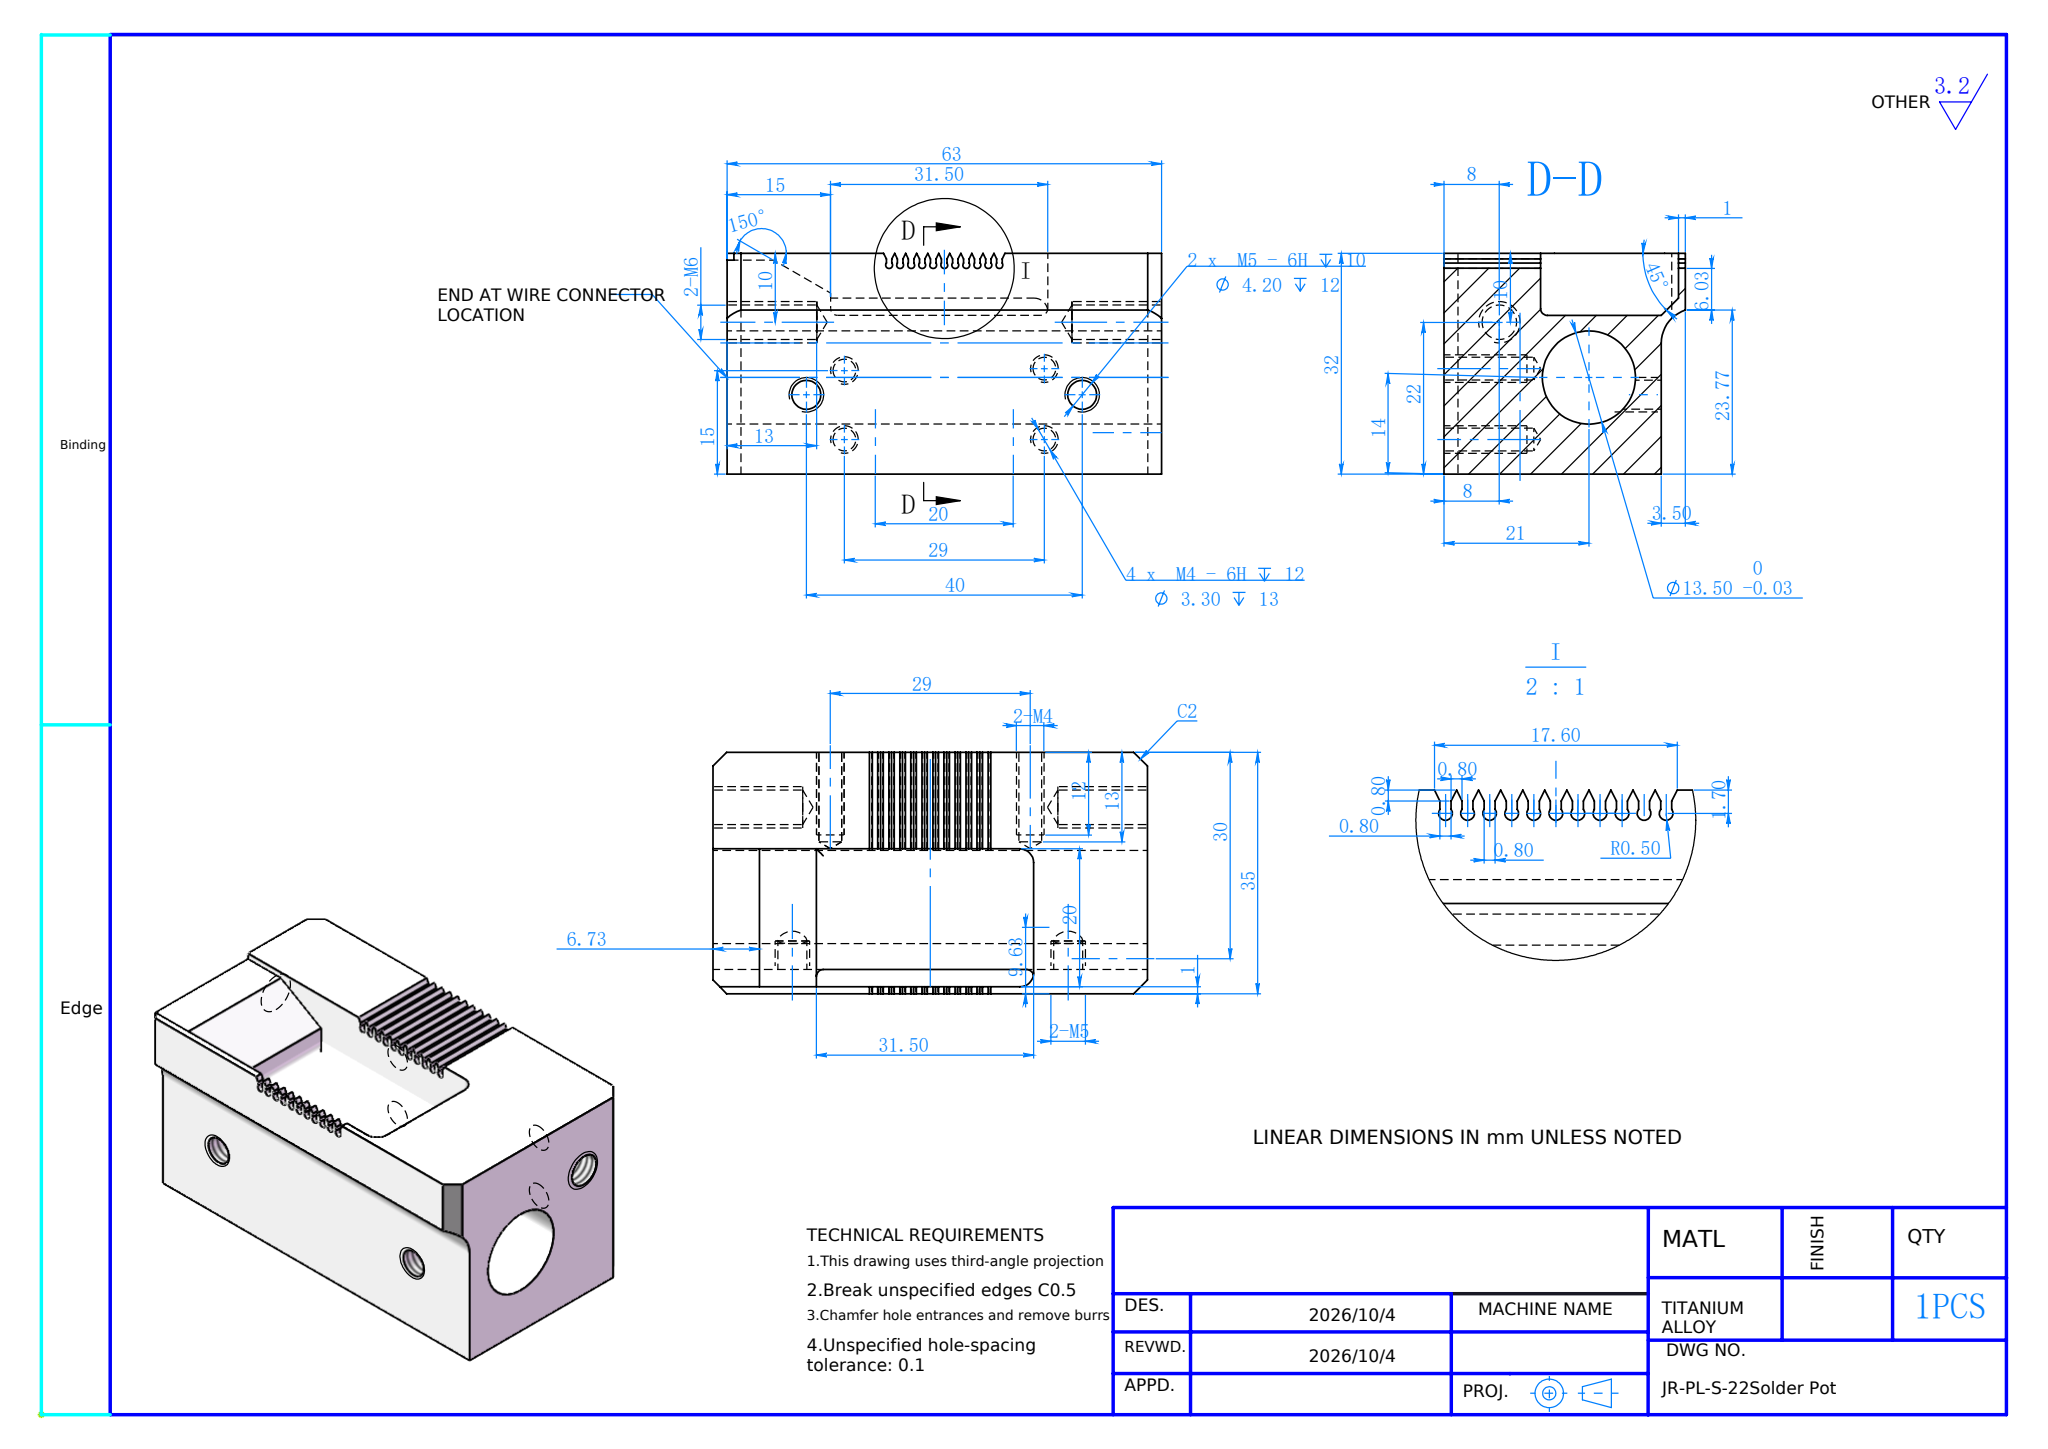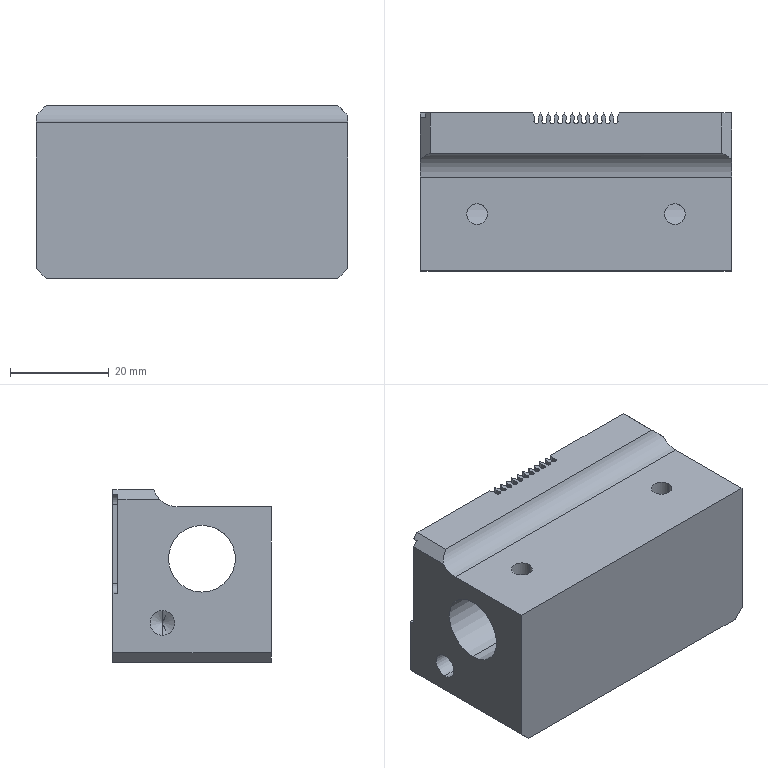Part | SolidWorks | mm | material TITANIUM ALLOY | 1 solid | 212 faces | box 63 x 32 x 35 mm | volume 48726 mm3 | plane 109 | cylinder 90 | cone 12 | torus 1 | commonest cylinder face diameters 1 x66 3.3 x8 5 x4 4.2 x4 2 x3 13.5 x2 4 x2 10 x1